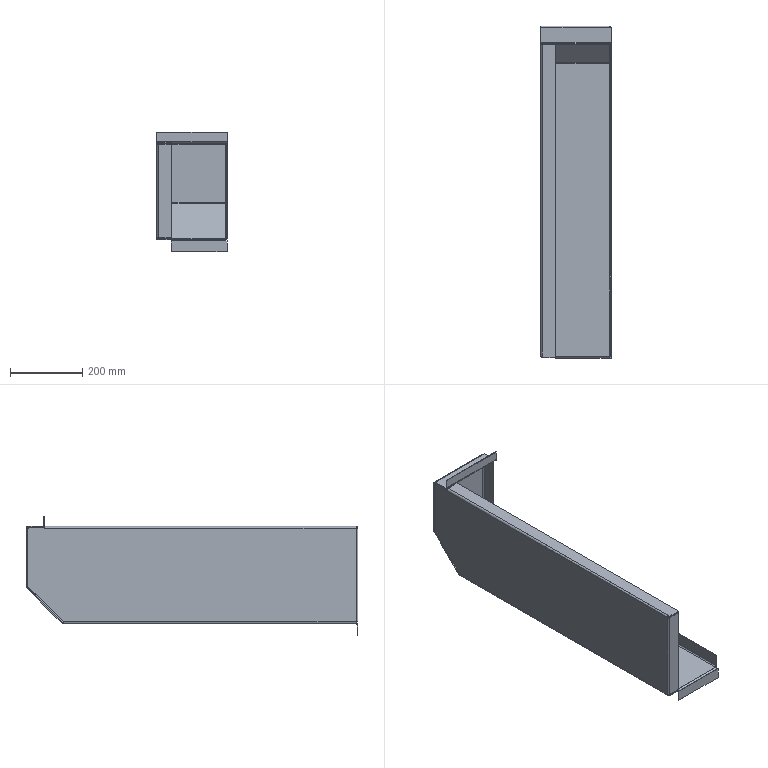Component | NX | SIDE_COLUMN_FRONT_RIGHT | 1 solid | 93 faces | volume 1115523 mm3 | plane 70 | cylinder 23 | commonest cylinder face diameters 6 x12 10 x11